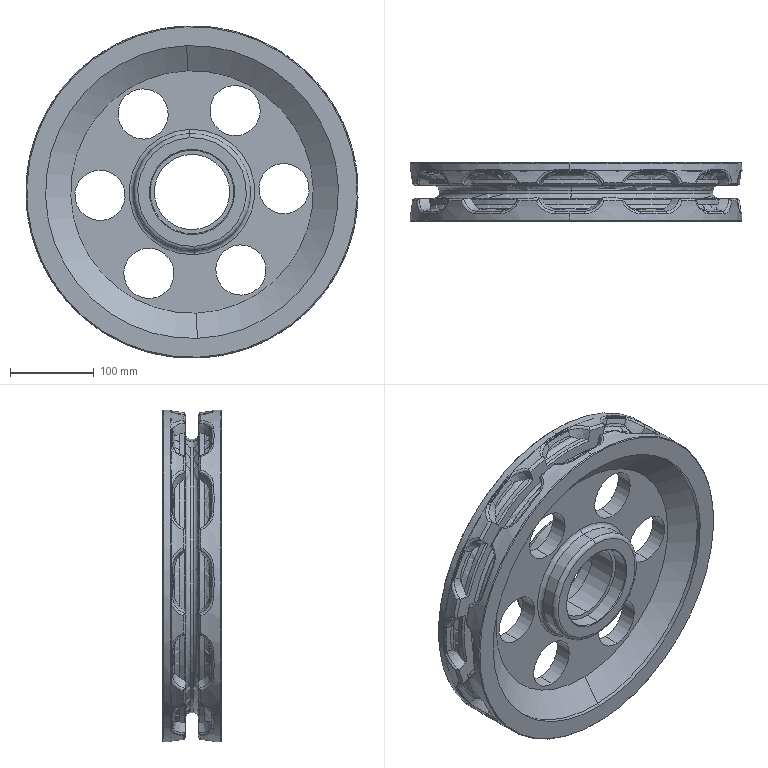Component | SolidWorks | LowerTensioningDeviceAssembly-1_DriveSprocket-DrivenWithBearingHole2-1 | 1 solid | 344 faces | volume 3491477 mm3 | cone 142 | spline 72 | cylinder 58 | torus 38 | plane 34 | commonest cylinder face diameters 367 x26 60 x12 100 x4 140 x4 350 x4 397 x4 90 x2 327 x2